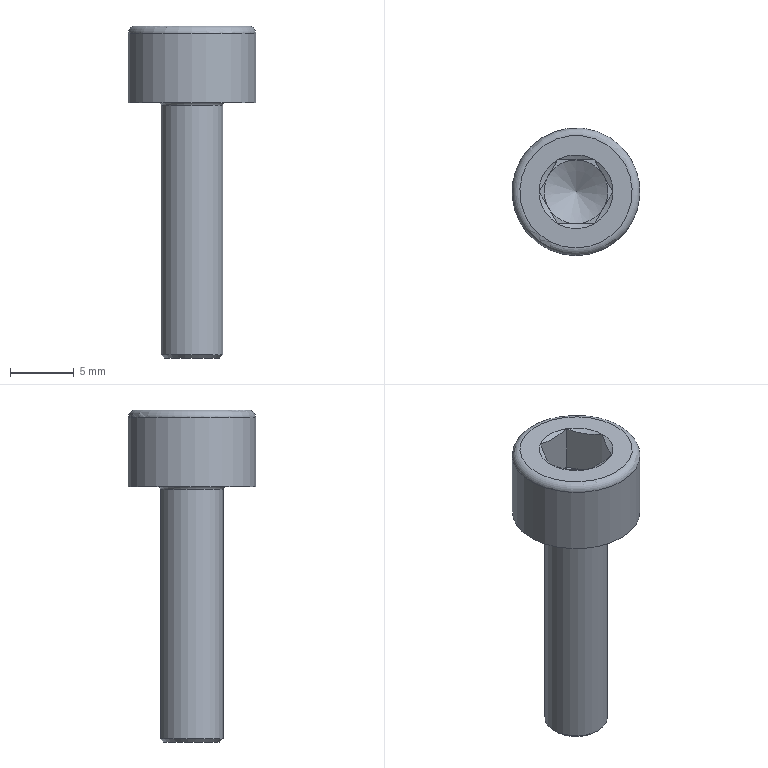Component | NX | SCREW_M6X20_2 | 1 solid | 27 faces | volume 754 mm3 | plane 15 | cone 8 | cylinder 2 | torus 2 | commonest cylinder face diameters 4.891 x1 10 x1